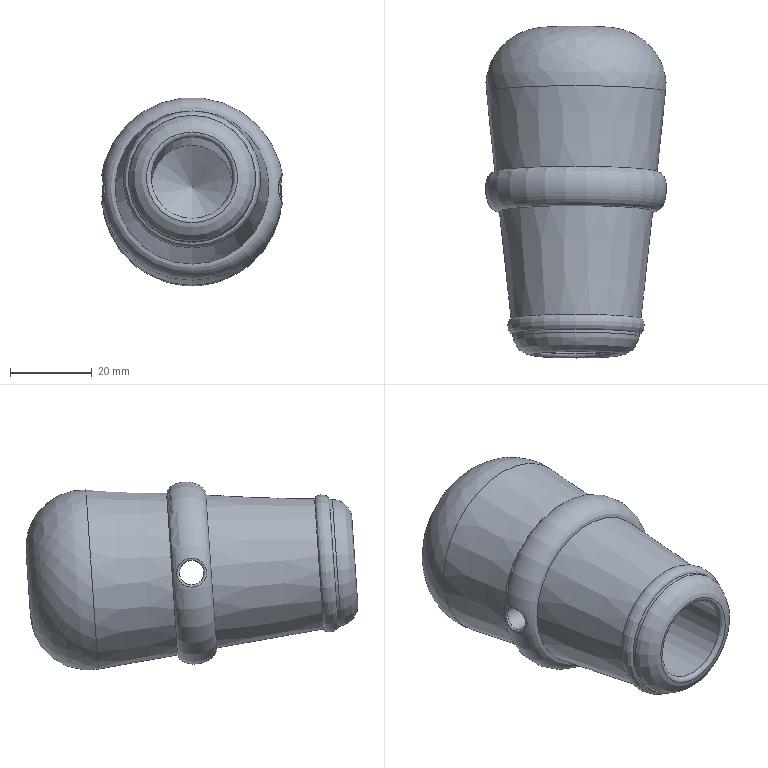Component | NX | BARREL | 1 solid | 17 faces | volume 79018 mm3 | cone 6 | spline 3 | cylinder 3 | other 2 | torus 2 | plane 1 | commonest cylinder face diameters 20 x1 8.5 x1 6 x1